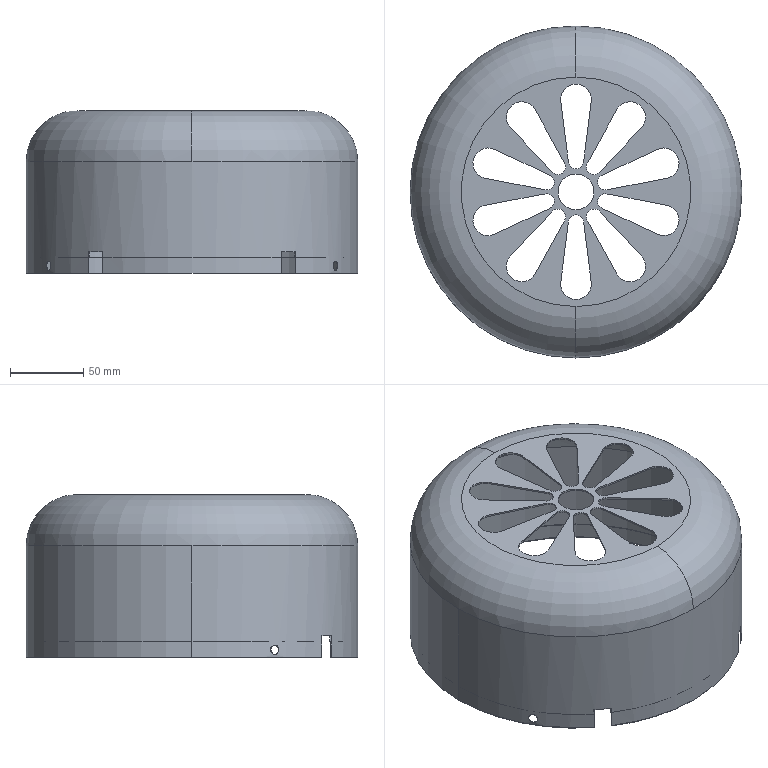Component | SolidWorks | Three-PhaseAsynchronousMotor-1_MotorProtectiveCover-1 | 1 solid | 88 faces | volume 99068 mm3 | cylinder 48 | plane 36 | torus 4 | commonest cylinder face diameters 21 x18 10.5 x14 6.3 x6 225.5 x4 226.642 x2 224.542 x2 24.5 x2